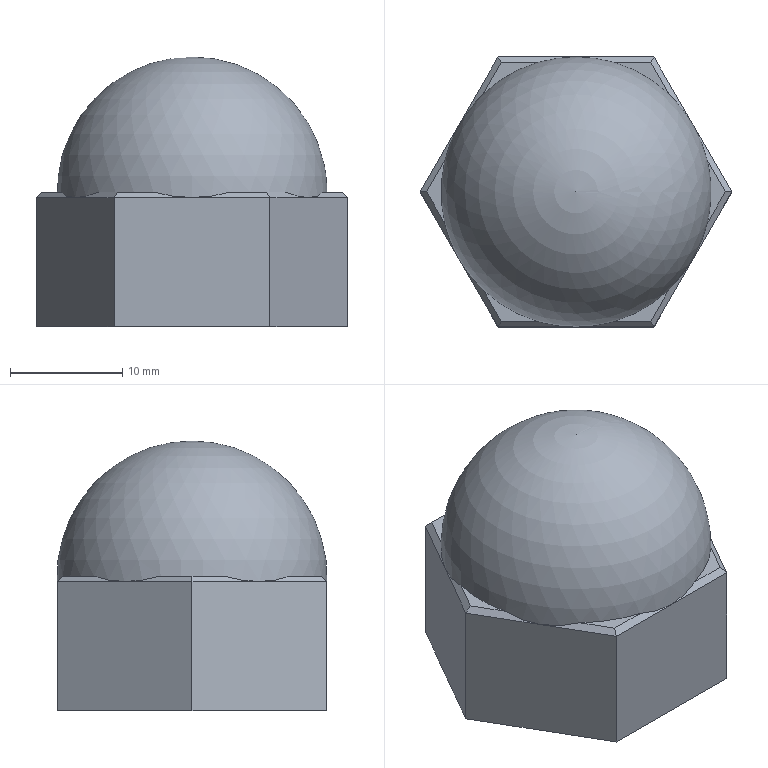Component | NX | NUT_CAP | 1 solid | 27 faces | volume 7028 mm3 | plane 21 | spline 3 | cylinder 2 | sphere 1 | commonest cylinder face diameters 16 x1 17 x1